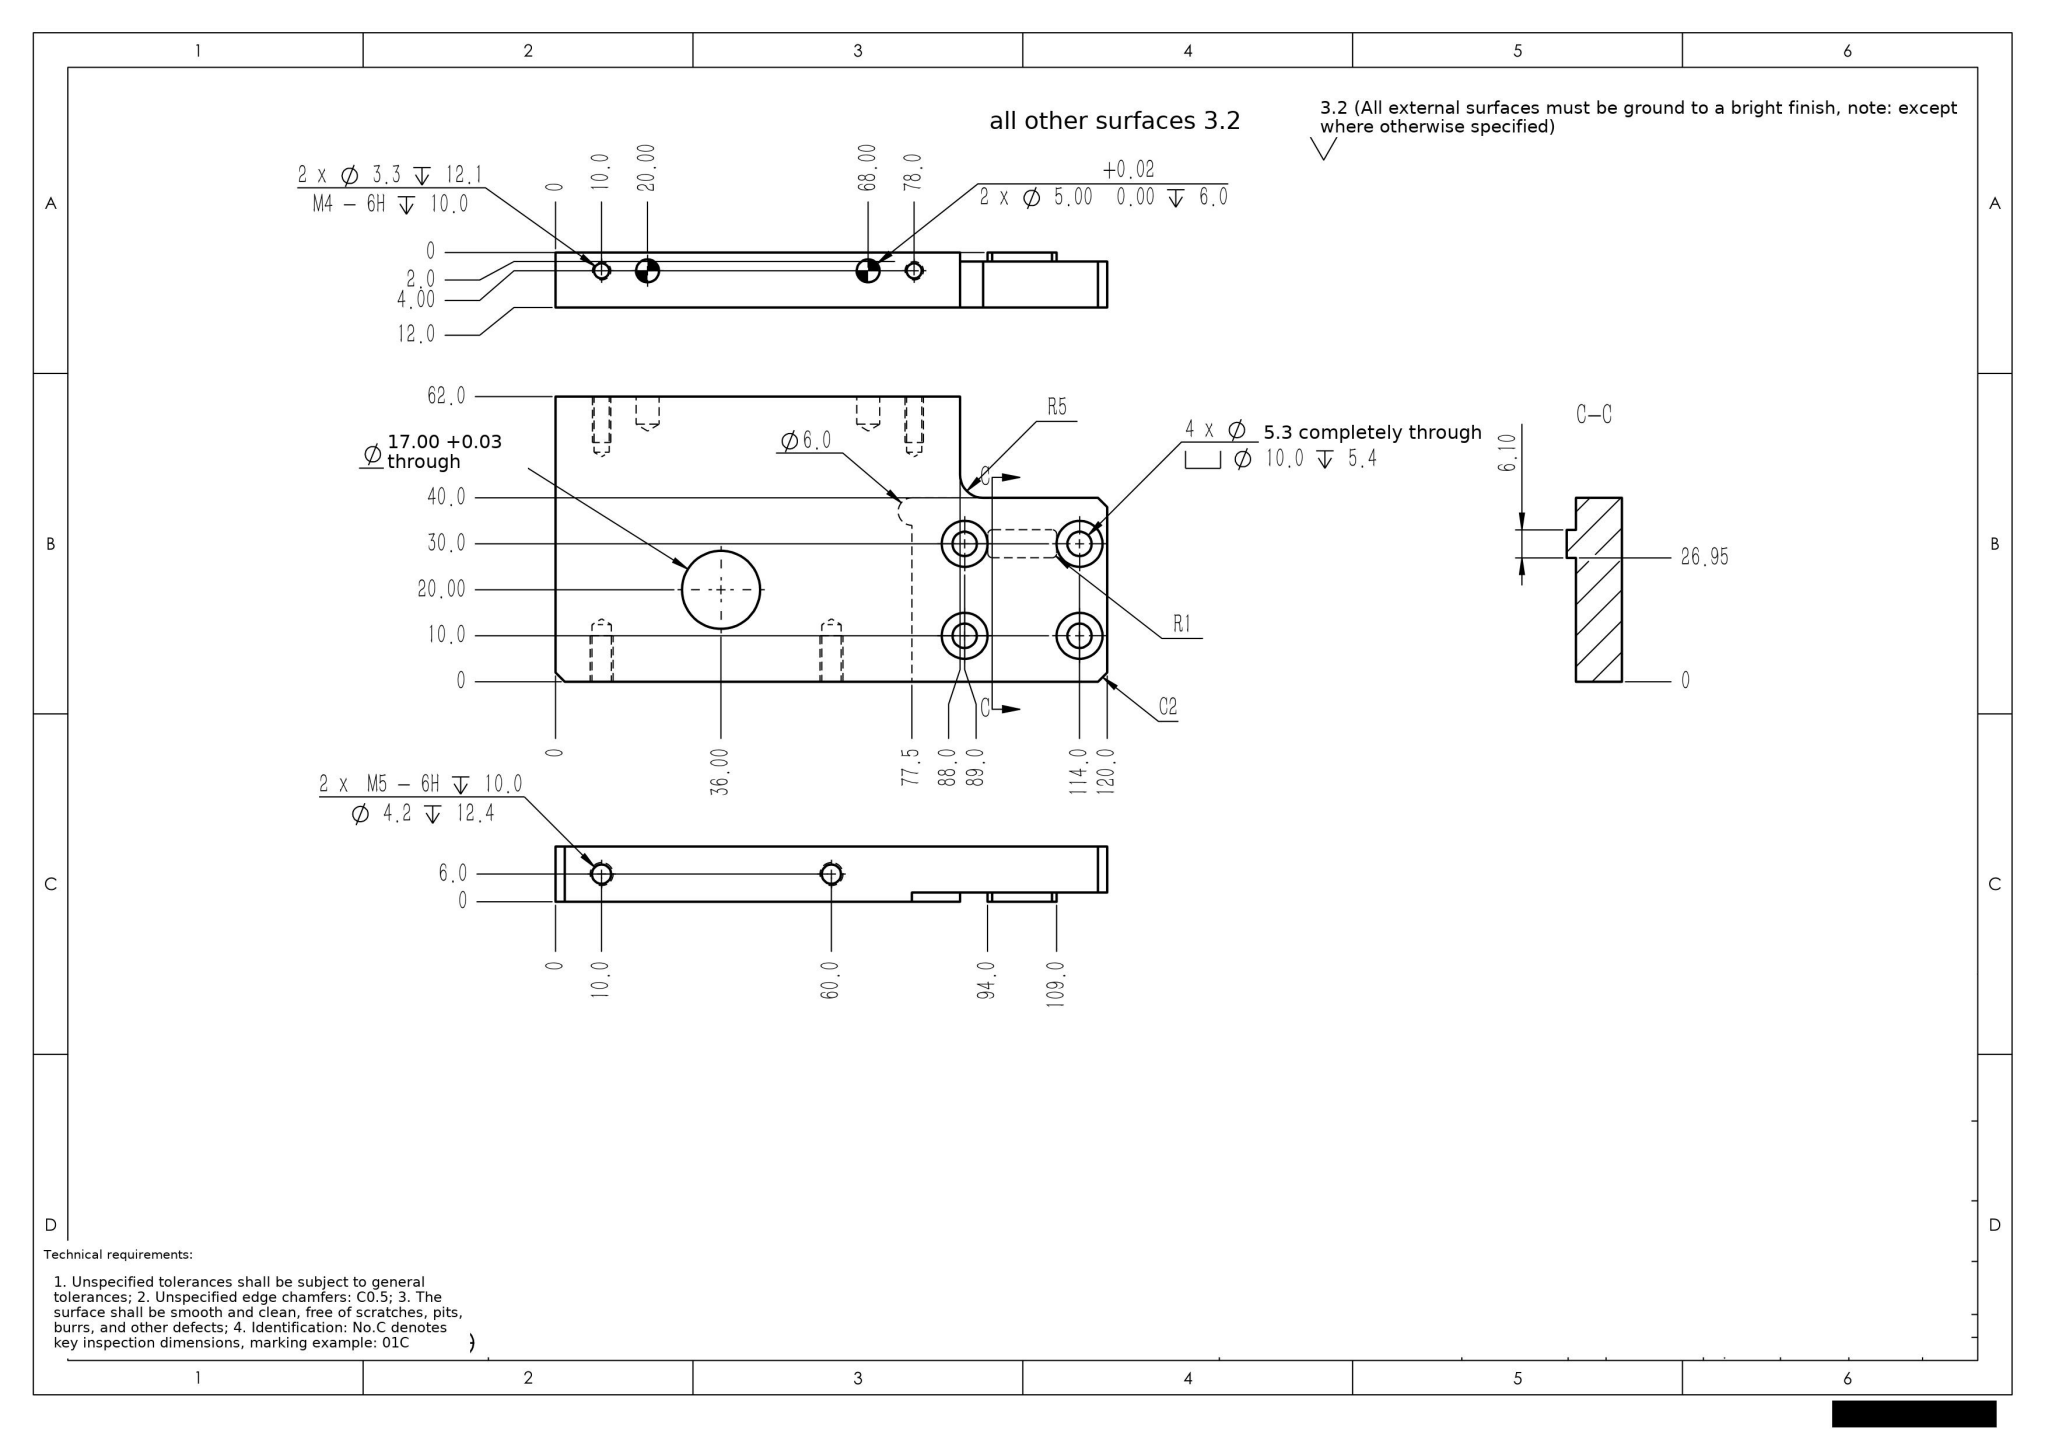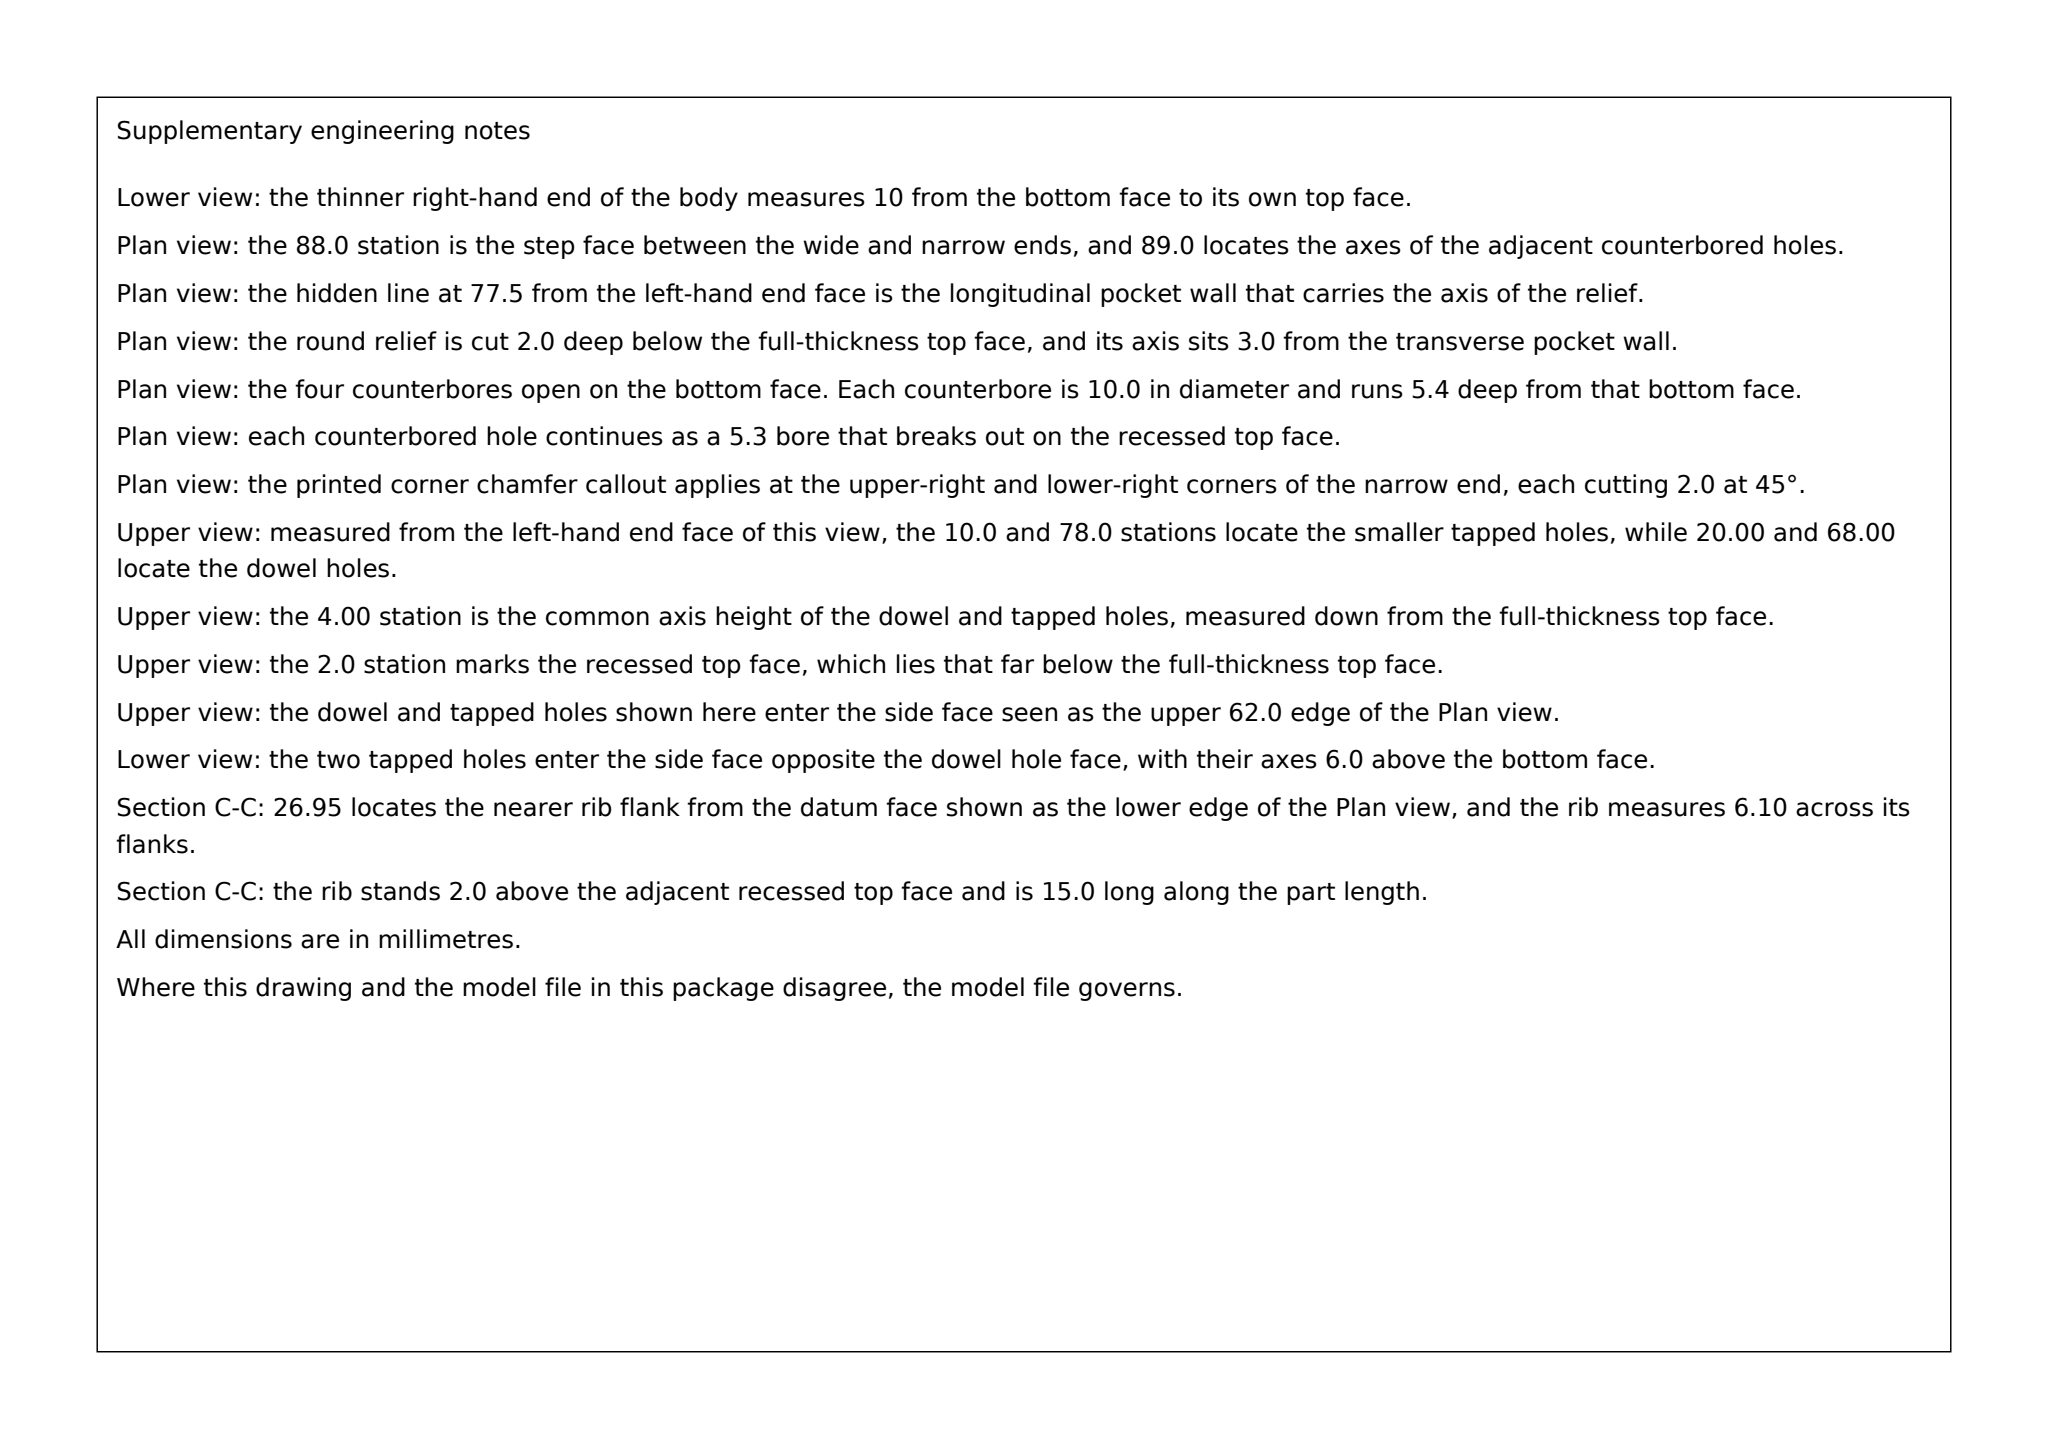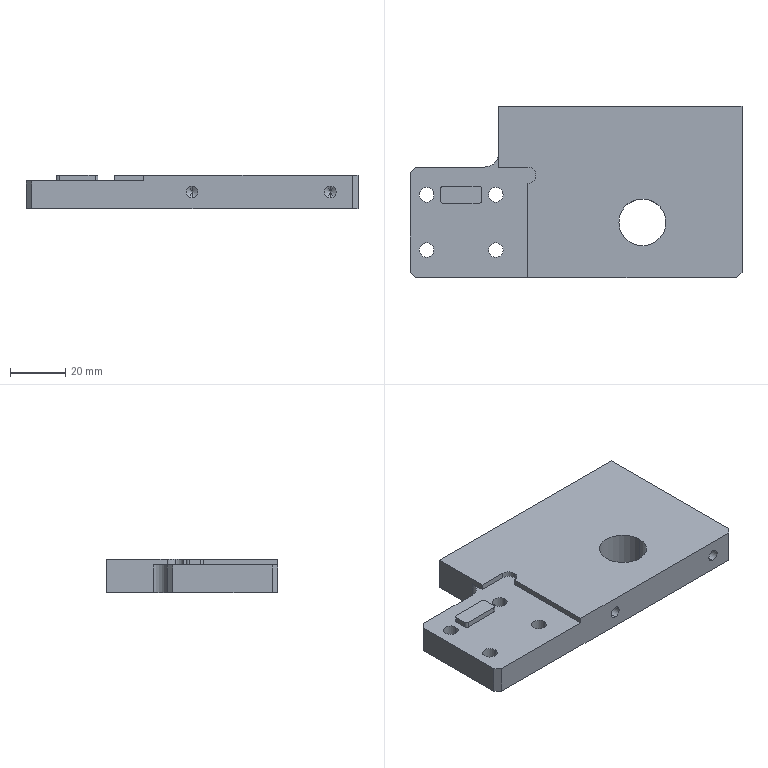Part | SolidWorks | mm | 1 solid | 72 faces | box 120 x 62 x 12 mm | volume 71925 mm3 | cylinder 37 | plane 23 | cone 12 | commonest cylinder face diameters 10 x9 5.3 x8 5 x4 3.3 x4 4.2 x4 2 x4 6 x2 17 x2
Drawing notes:
Ø6.0 NOTCH CL 37.0 FROM BOTTOM EDGE (3.0 BELOW 40.0 FACE) | from the solid: cyl dia 6.0 axis z at [42.5,37.0]; y-planes at 0.0 and 40.0
Ø6.0 NOTCH DP 2.0 FROM TOP FACE (Z 10.0 TO 12.0) | from the solid: cyl dia 6.0 length 2.0; z-planes 10.0 and 12.0, bbox z=12.0
build123d program:
from build123d import *

# Parameters (mm, degrees)
SKETCH1_W                                       = 120
SKETCH1_H                                       = 40
BOSS_EXTRUDE1_DEPTH                             = 12
SKETCH2_R                                       = 8.5
CUT_EXTRUDE1_DEPTH                              = 65.374
SKETCH7_W                                       = 32
SKETCH7_H                                       = 2
CUT_EXTRUDE4_DEPTH                              = 74.103
M5_HEX_SOCKET_HEAD_CAP_SCREW_CBORE1_D           = 5.3
M5_HEX_SOCKET_HEAD_CAP_SCREW_CBORE1_CBORE_D     = 10
M5_HEX_SOCKET_HEAD_CAP_SCREW_CBORE1_CBORE_DEPTH = 5.4
SKETCH12_W                                      = 15
SKETCH12_H                                      = 6.1
BOSS_EXTRUDE2_DEPTH                             = 2
M5_TAPPED_HOLE1_D                               = 4.2
M5_TAPPED_HOLE1_DEPTH                           = 12.4
M5_TAPPED_HOLE1_TIP                             = 1.262
SKETCH15_W                                      = 88
SKETCH15_H                                      = 12
BOSS_EXTRUDE3_DEPTH                             = 22
M4_TAPPED_HOLE1_D                               = 3.3
M4_TAPPED_HOLE1_DEPTH                           = 12.1
M4_TAPPED_HOLE1_TIP                             = 0.9914
SIZE_MM_DOWEL_PIN_HOLE_1_D                      = 5
SIZE_MM_DOWEL_PIN_HOLE_1_DEPTH                  = 6
SIZE_MM_DOWEL_PIN_HOLE_1_TIP                    = 1.502
SKETCH21_W                                      = 10.5
SKETCH21_H                                      = 40
CUT_EXTRUDE6_DEPTH                              = 2
SKETCH22_R                                      = 3
CUT_EXTRUDE7_DEPTH                              = 2
FILLET3_R                                       = 5
CHAMFER1_SIZE                                   = 2
FILLET2_R                                       = 1


with BuildPart() as part:
    # Sketch1 → Boss-Extrude1 (new body)
    with BuildSketch(Plane.XY):
        Rectangle(SKETCH1_W, SKETCH1_H)
    extrude(amount=BOSS_EXTRUDE1_DEPTH)

    # Sketch2 → Cut-Extrude1 (cut, through all)
    with BuildSketch(Plane.XY.offset(12)):
        with Locations((24, 0)):
            Circle(SKETCH2_R)
    extrude(amount=-CUT_EXTRUDE1_DEPTH, mode=Mode.SUBTRACT)

    # Sketch7 → Cut-Extrude4 (cut, through all)
    with BuildSketch(Plane(origin=(0, 20, 0), x_dir=(1, 0, 0), z_dir=(0, 1, 0))):
        with Locations((-44, -11)):
            Rectangle(SKETCH7_W, SKETCH7_H)
    extrude(amount=-CUT_EXTRUDE4_DEPTH, mode=Mode.SUBTRACT)

    # M5 Hex Socket Head Cap Screw CBORE1 (through all)
    with Locations(Plane(origin=(0, 0, 0), x_dir=(-1, 0, 0), z_dir=(0, 0, -1))):
        with Locations((54, -10), (29, -10), (29, 10), (54, 10)):
            CounterBoreHole(M5_HEX_SOCKET_HEAD_CAP_SCREW_CBORE1_D / 2, M5_HEX_SOCKET_HEAD_CAP_SCREW_CBORE1_CBORE_D / 2, M5_HEX_SOCKET_HEAD_CAP_SCREW_CBORE1_CBORE_DEPTH)

    # Sketch12 → Boss-Extrude2 (add)
    with BuildSketch(Plane.XY.offset(10)):
        with Locations((-41.5, 10)):
            Rectangle(SKETCH12_W, SKETCH12_H)
    extrude(amount=BOSS_EXTRUDE2_DEPTH)

    # M5 Tapped Hole1
    with Locations(Plane(origin=(0, -20, 0), x_dir=(-1, 0, 0), z_dir=(0, -1, 0))):
        with Locations((-50, -6), (0, -6)):
            Hole(M5_TAPPED_HOLE1_D / 2, depth=M5_TAPPED_HOLE1_DEPTH)
            with Locations((0, 0, -(M5_TAPPED_HOLE1_DEPTH + M5_TAPPED_HOLE1_TIP / 2))):  # 118° drill point
                Cone(0, M5_TAPPED_HOLE1_D / 2, M5_TAPPED_HOLE1_TIP, mode=Mode.SUBTRACT)

    # Sketch15 → Boss-Extrude3 (add)
    with BuildSketch(Plane(origin=(0, 20, 0), x_dir=(1, 0, 0), z_dir=(0, 1, 0))):
        with Locations((16, -6)):
            Rectangle(SKETCH15_W, SKETCH15_H)
    extrude(amount=BOSS_EXTRUDE3_DEPTH)

    # M4 Tapped Hole1
    with Locations(Plane(origin=(0, 42, 0), x_dir=(1, 0, 0), z_dir=(0, 1, 0))):
        with Locations((50, -8), (-18, -8)):
            Hole(M4_TAPPED_HOLE1_D / 2, depth=M4_TAPPED_HOLE1_DEPTH)
            with Locations((0, 0, -(M4_TAPPED_HOLE1_DEPTH + M4_TAPPED_HOLE1_TIP / 2))):  # 118° drill point
                Cone(0, M4_TAPPED_HOLE1_D / 2, M4_TAPPED_HOLE1_TIP, mode=Mode.SUBTRACT)

    # Size mm Dowel Pin Hole 1
    with Locations(Plane(origin=(0, 42, 0), x_dir=(1, 0, 0), z_dir=(0, 1, 0))):
        with Locations((-8, -8), (40, -8)):
            Hole(SIZE_MM_DOWEL_PIN_HOLE_1_D / 2, depth=SIZE_MM_DOWEL_PIN_HOLE_1_DEPTH)
            with Locations((0, 0, -(SIZE_MM_DOWEL_PIN_HOLE_1_DEPTH + SIZE_MM_DOWEL_PIN_HOLE_1_TIP / 2))):  # 118° drill point
                Cone(0, SIZE_MM_DOWEL_PIN_HOLE_1_D / 2, SIZE_MM_DOWEL_PIN_HOLE_1_TIP, mode=Mode.SUBTRACT)

    # Sketch21 → Cut-Extrude6 (cut)
    with BuildSketch(Plane.XY.offset(12)):
        with Locations((-22.75, 0)):
            Rectangle(SKETCH21_W, SKETCH21_H)
    extrude(amount=-CUT_EXTRUDE6_DEPTH, mode=Mode.SUBTRACT)

    # Sketch22 → Cut-Extrude7 (cut)
    with BuildSketch(Plane.XY.offset(12)):
        with Locations((-17.5, 17)):
            Circle(SKETCH22_R)
    extrude(amount=-CUT_EXTRUDE7_DEPTH, mode=Mode.SUBTRACT)

    # Fillet3
    fillet3_edges = [part.edges().sort_by_distance(p)[0] for p in [
        (-28, 20, 5),
    ]]
    fillet(fillet3_edges, radius=FILLET3_R)

    # Chamfer1
    chamfer1_edges = [part.edges().sort_by_distance(p)[0] for p in [
        (-60, -20, 5),
        (-60, 20, 5),
        (60, -20, 6),
    ]]
    chamfer(chamfer1_edges, length=CHAMFER1_SIZE)

    # Fillet2
    fillet2_edges = [part.edges().sort_by_distance(p)[0] for p in [
        (-49, 6.95, 11),
        (-49, 13.05, 11),
        (-34, 13.05, 11),
        (-34, 6.95, 11),
    ]]
    fillet(fillet2_edges, radius=FILLET2_R)


solid = part.part